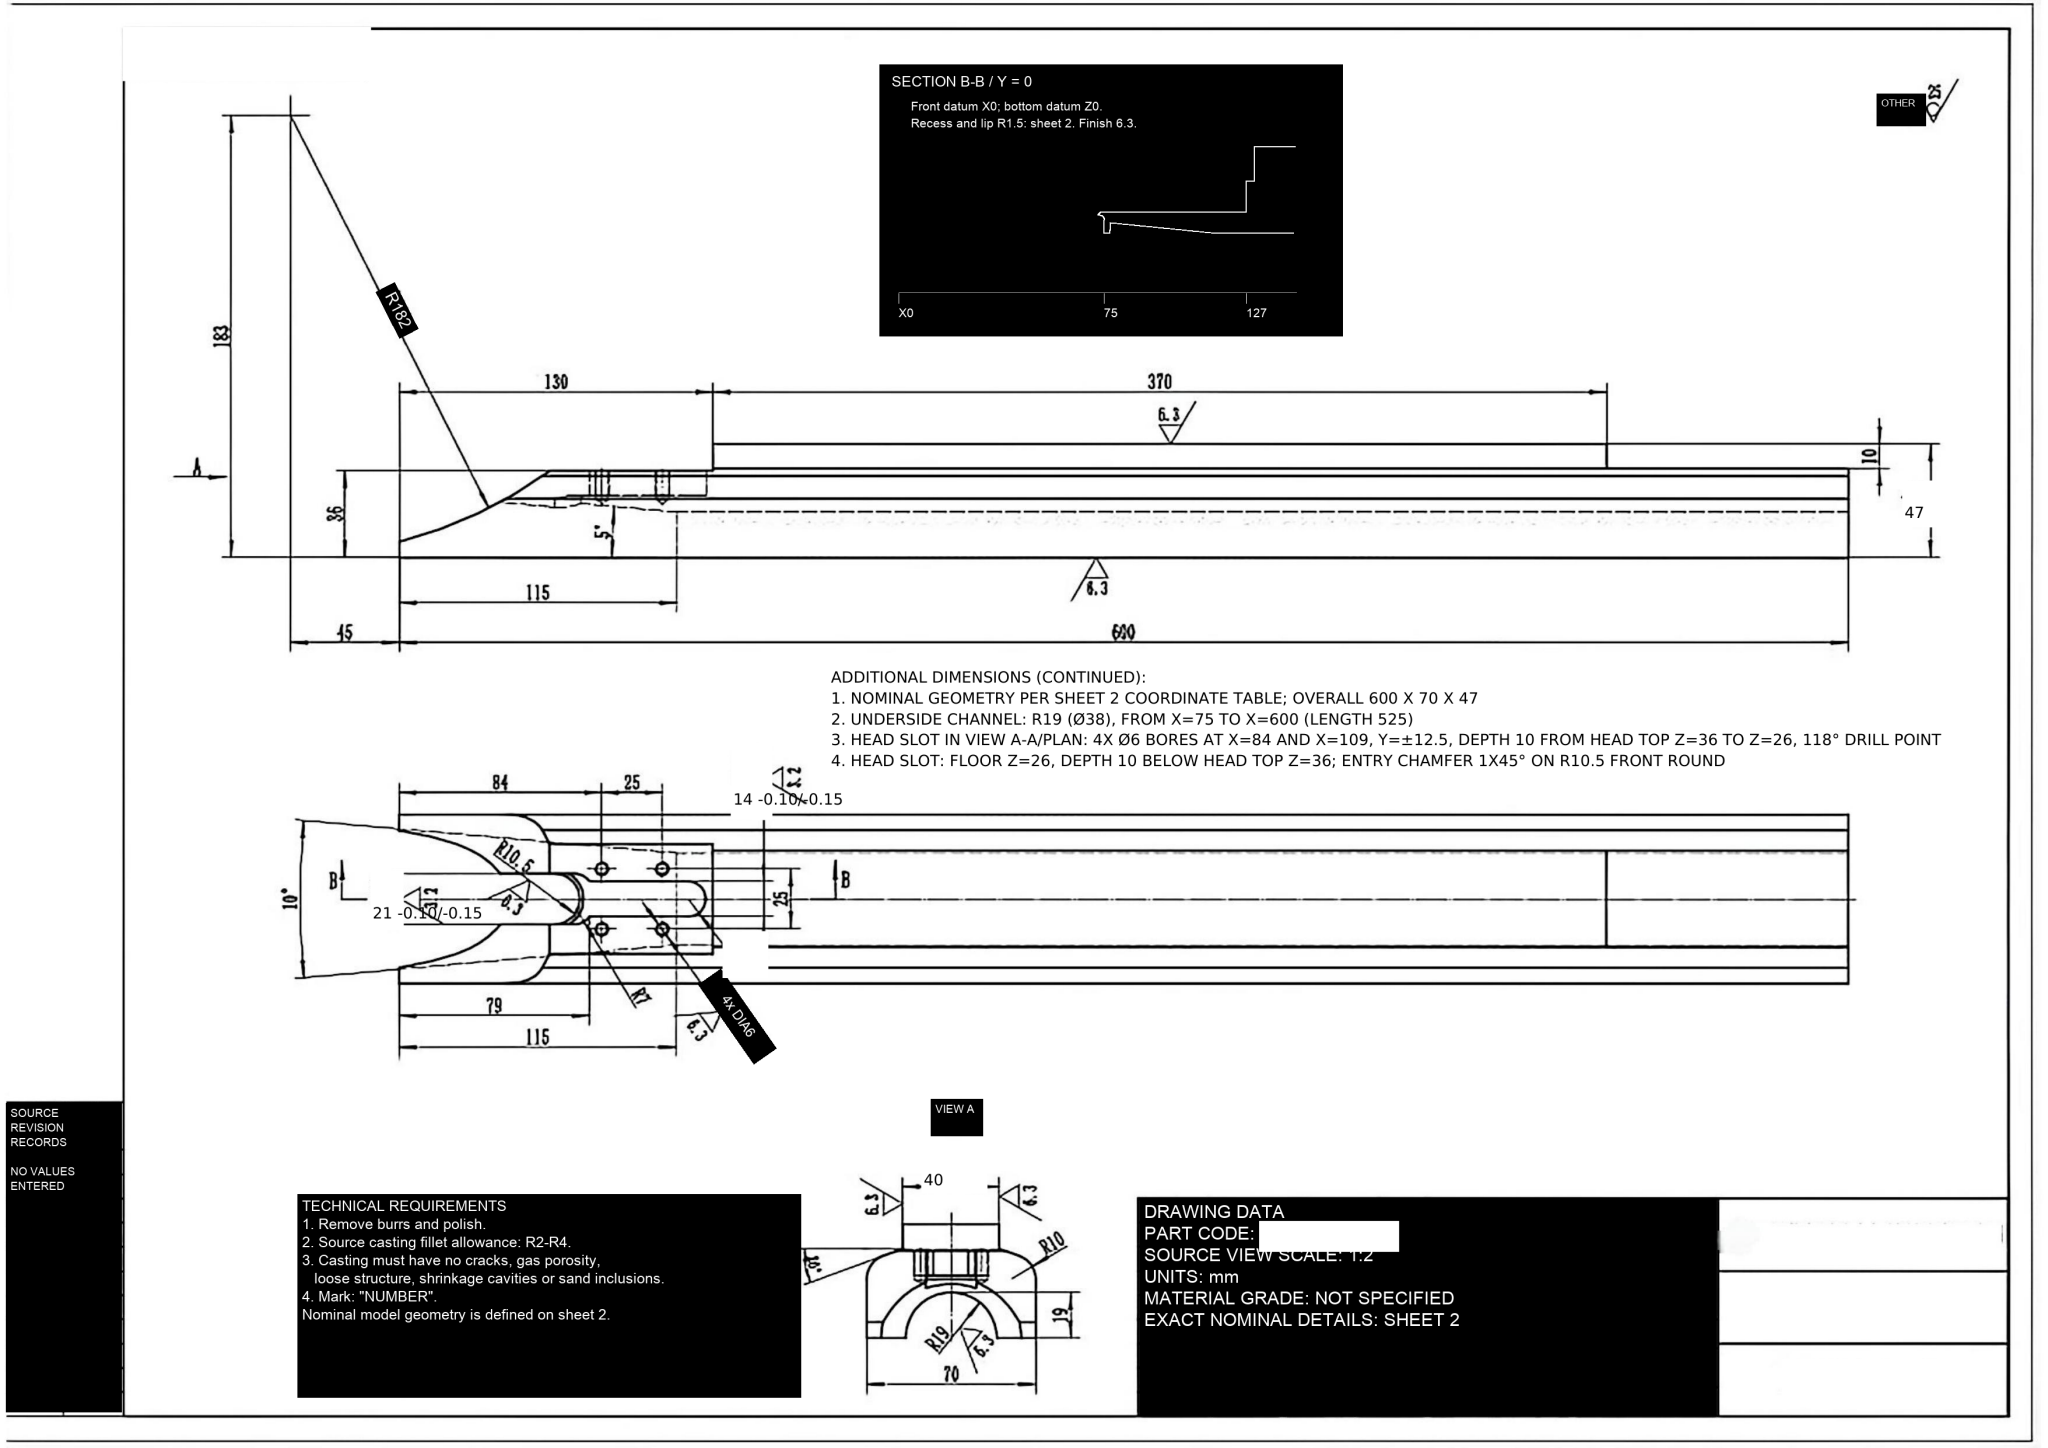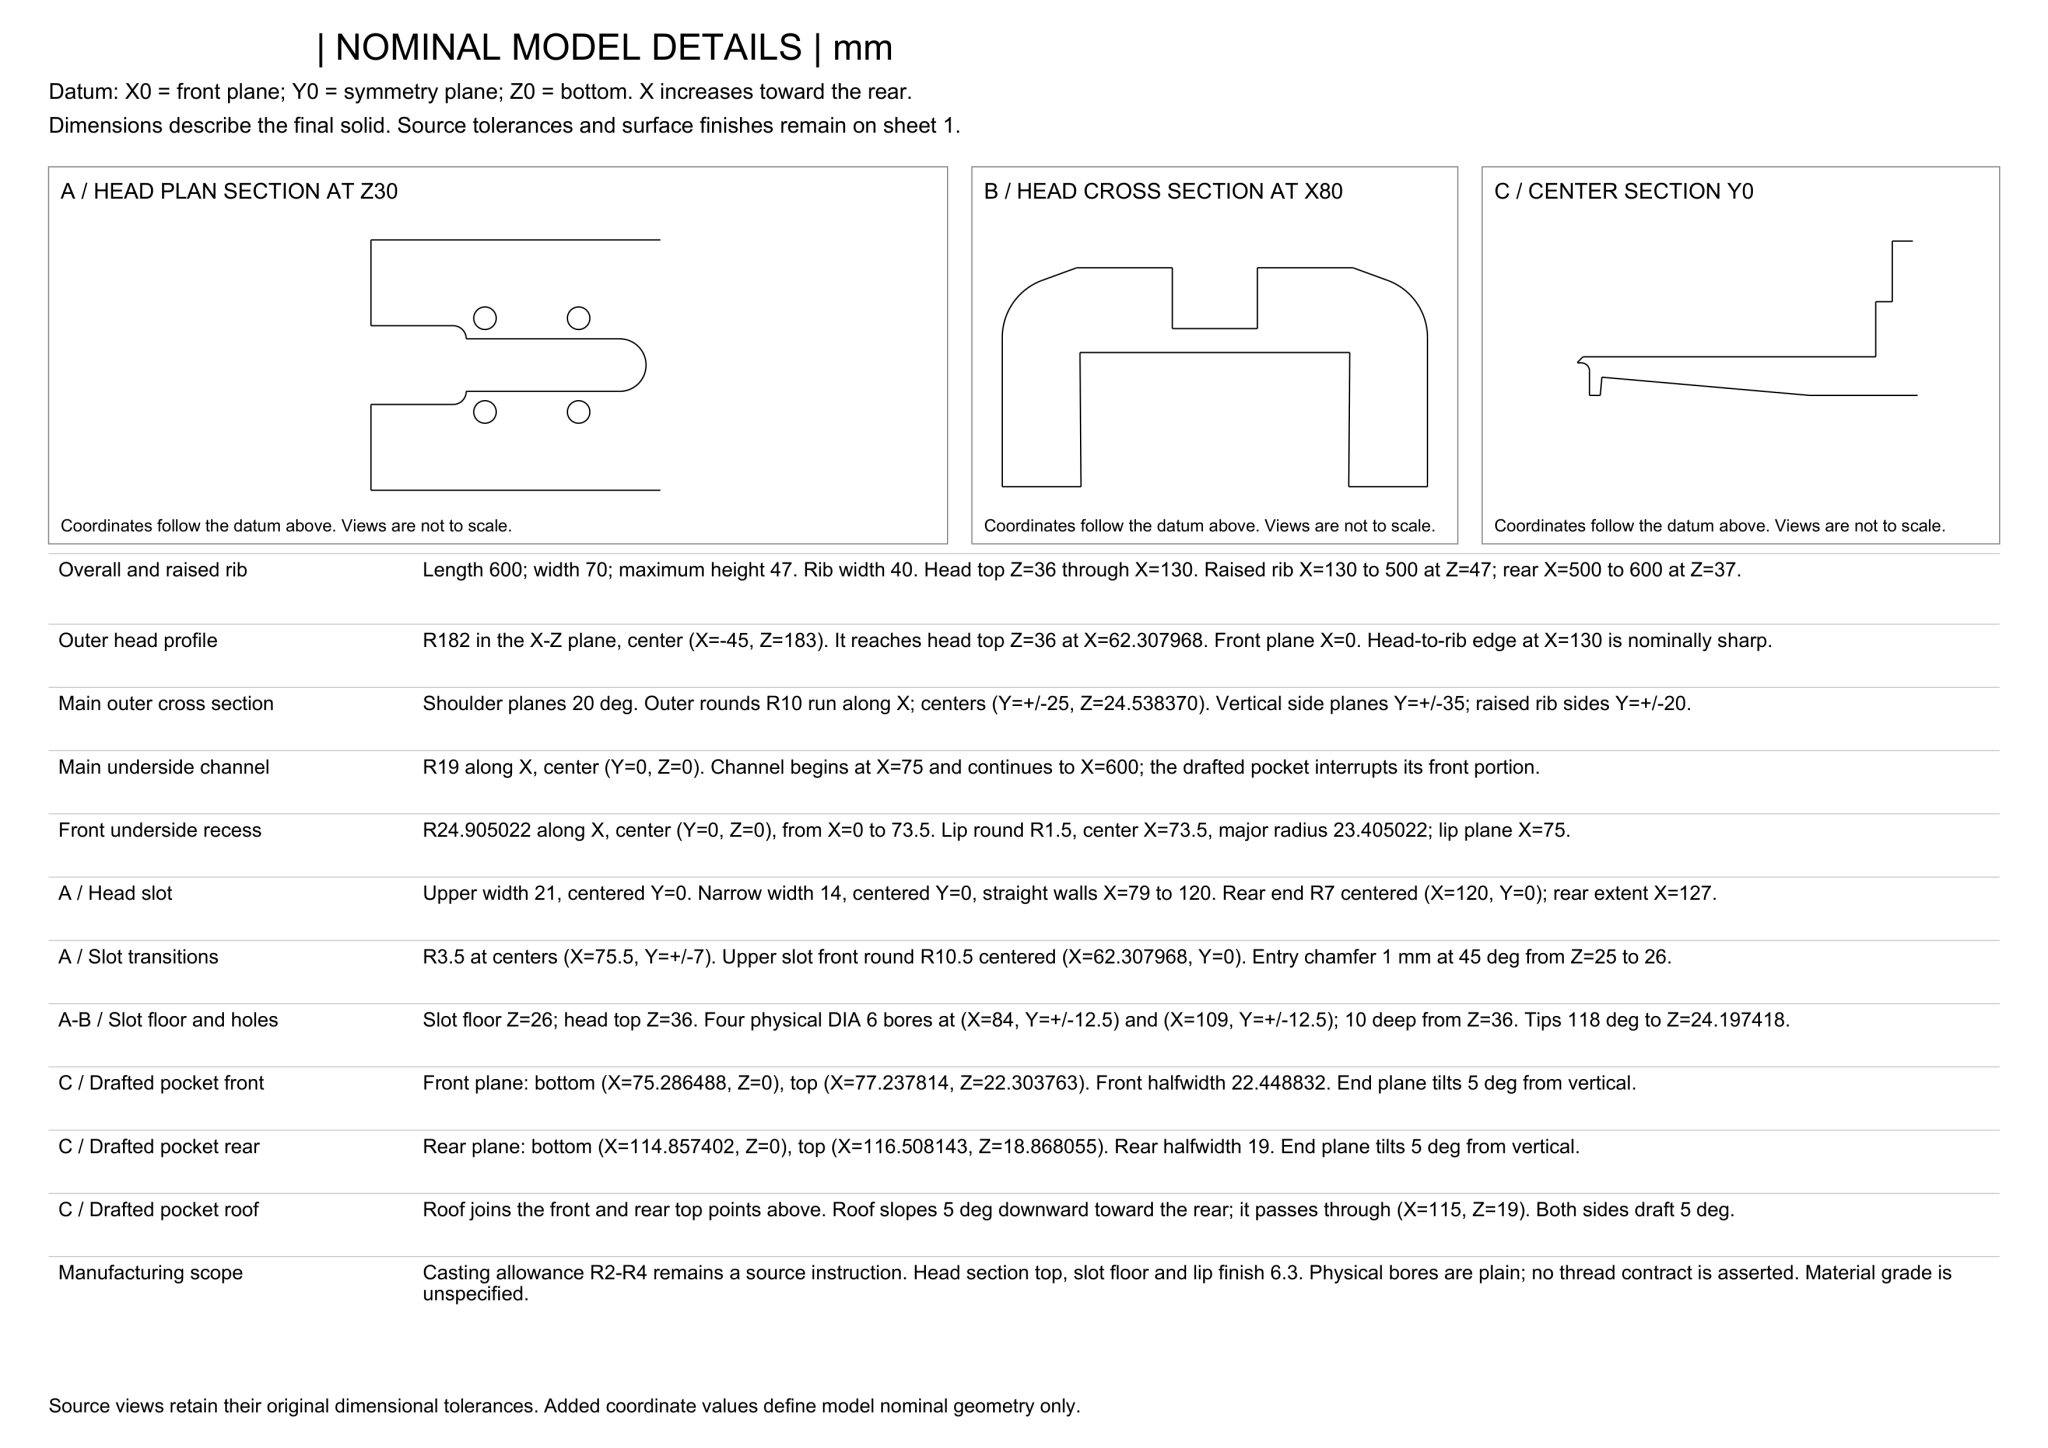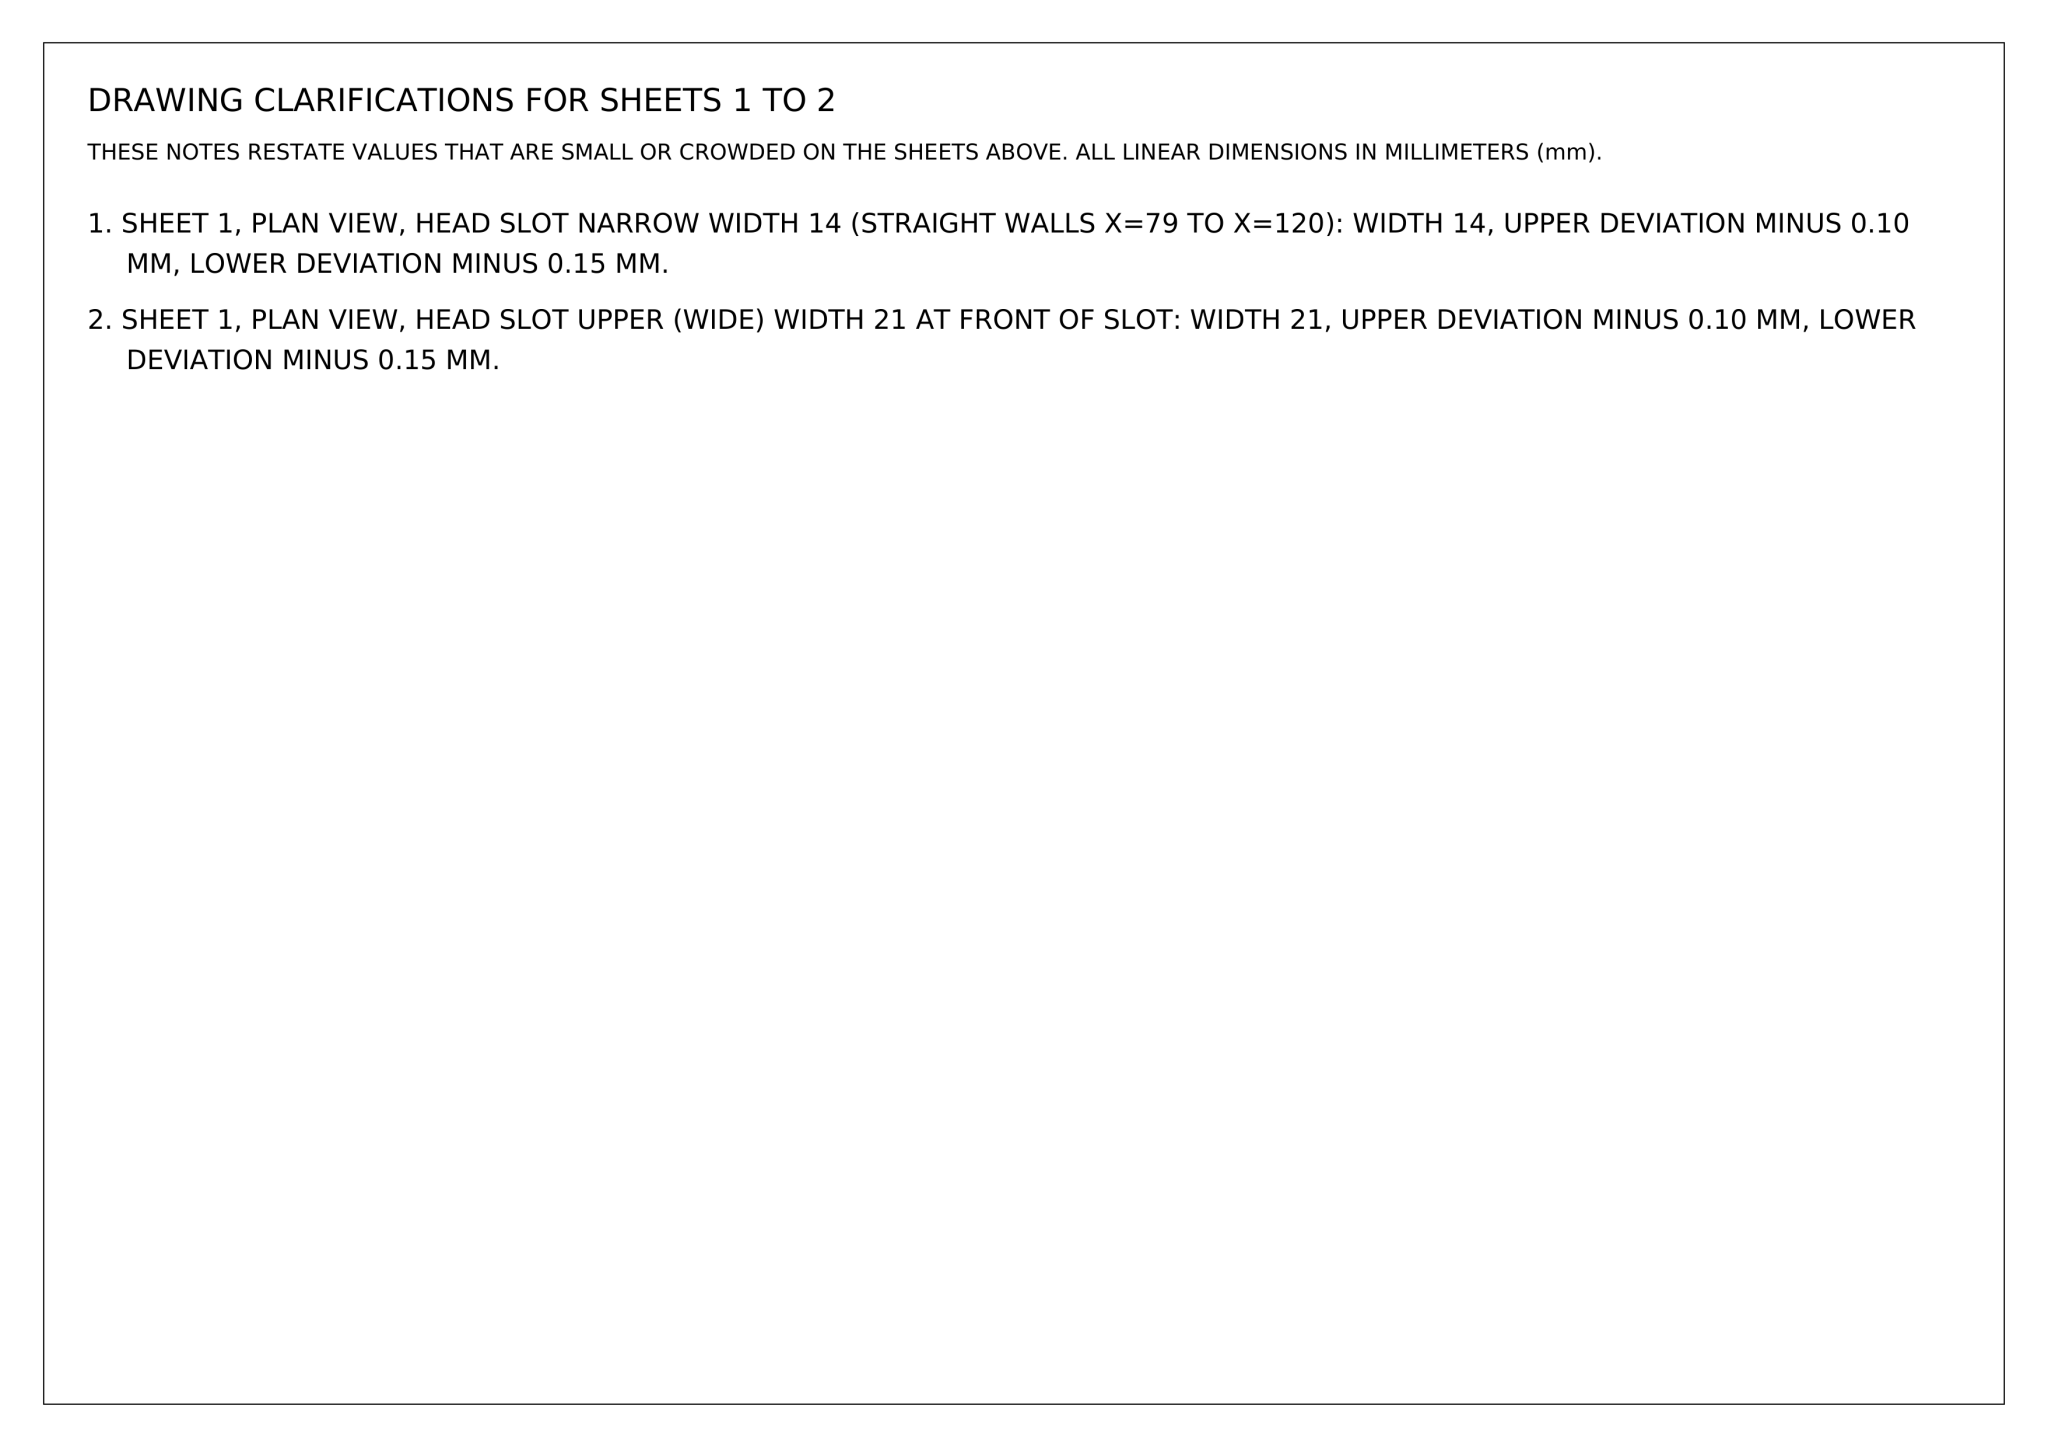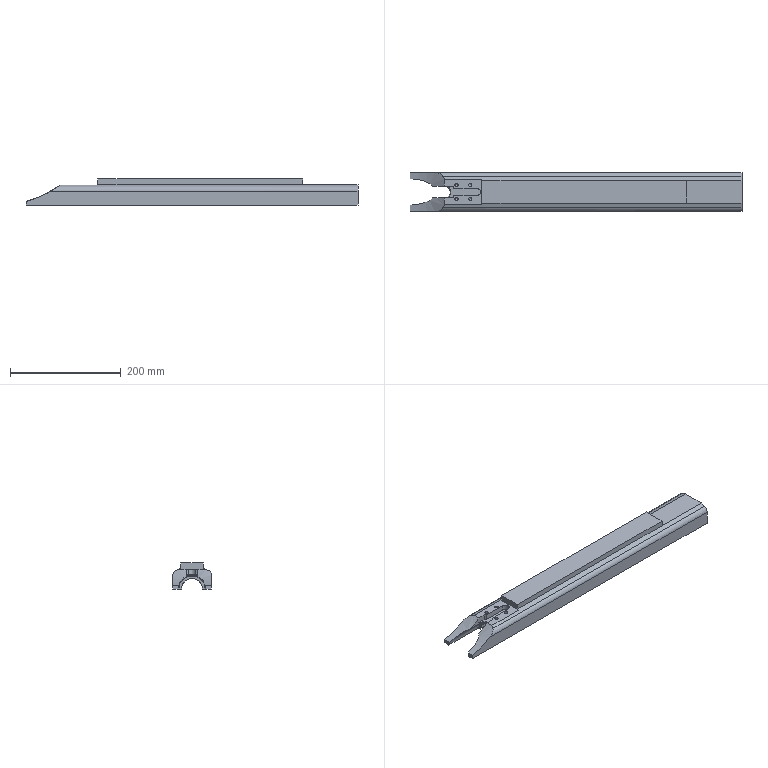Part | NX | mm | 1 solid | 49 faces | box 600 x 70 x 47 mm | volume 1184615 mm3 | plane 28 | cylinder 15 | cone 5 | torus 1 | commonest cylinder face diameters 6 x4 38 x2 364 x2 20 x2 7 x2 21 x1 14 x1 49.81 x1